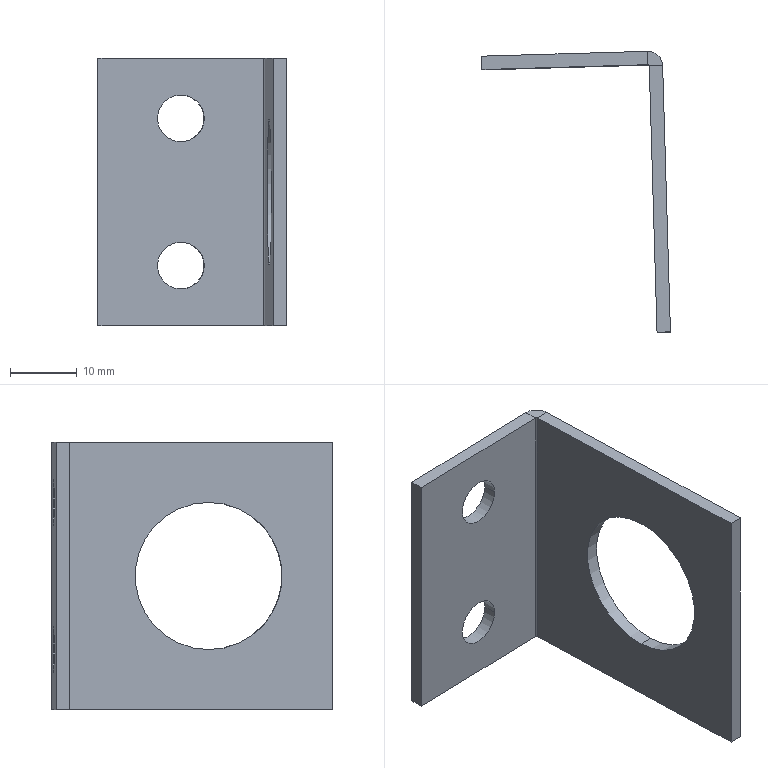Component | SolidWorks | CylinderFixingSheetMetal-1 | 1 solid | 20 faces | box 28.21 x 41.98 x 40 mm | volume 4405 mm3 | plane 12 | cylinder 8 | commonest cylinder face diameters 7 x4 22 x2 4.4 x1 0.4 x1 | material Q235
STEP:
#1=CARTESIAN_POINT('',(-7.163,-7.612,-48.827));
#2=VERTEX_POINT('',#1);
#3=CARTESIAN_POINT('',(-6.887,-7.604,-48.827));
#4=VERTEX_POINT('',#3);
#5=CARTESIAN_POINT('',(-7.025,-7.608,-48.827));
#6=DIRECTION('',(0.02918,-0.9996,-0.));
#7=DIRECTION('',(0.9996,0.02918,0.));
#8=AXIS2_PLACEMENT_3D('',#5,#6,#7);
#9=CIRCLE('',#8,0.1378);
#10=EDGE_CURVE('',#2,#4,#9,.T.);
#11=ORIENTED_EDGE('',*,*,#10,.T.);
#12=CARTESIAN_POINT('',(-6.89,-7.525,-48.827));
#13=VERTEX_POINT('',#12);
#14=CARTESIAN_POINT('',(-6.841,-9.178,-48.827));
#15=DIRECTION('',(-0.02918,0.9996,0.));
#16=VECTOR('',#15,39.37);
#17=LINE('',#14,#16);
#18=EDGE_CURVE('',#4,#13,#17,.T.);
#19=ORIENTED_EDGE('',*,*,#18,.T.);
#20=CARTESIAN_POINT('',(-7.165,-7.533,-48.827));
#21=VERTEX_POINT('',#20);
#22=CARTESIAN_POINT('',(-7.027,-7.529,-48.827));
#23=DIRECTION('',(-0.02918,0.9996,0.));
#24=DIRECTION('',(-0.9996,-0.02918,0.));
#25=AXIS2_PLACEMENT_3D('',#22,#23,#24);
#26=CIRCLE('',#25,0.1378);
#27=EDGE_CURVE('',#13,#21,#26,.T.);
#28=ORIENTED_EDGE('',*,*,#27,.T.);
#29=CARTESIAN_POINT('',(-7.117,-9.186,-48.827));
#30=DIRECTION('',(-0.02918,0.9996,0.));
#31=VECTOR('',#30,39.37);
#32=LINE('',#29,#31);
#33=EDGE_CURVE('',#2,#21,#32,.T.);
#34=ORIENTED_EDGE('',*,*,#33,.F.);
#35=EDGE_LOOP('',(#11,#19,#28,#34));
#36=FACE_OUTER_BOUND('',#35,.T.);
#37=CARTESIAN_POINT('',(-6.979,-9.182,-48.827));
#38=DIRECTION('',(-0.02918,0.9996,0.));
#39=DIRECTION('',(-0.9996,-0.02918,0.));
#40=AXIS2_PLACEMENT_3D('',#37,#38,#39);
#41=CYLINDRICAL_SURFACE('',#40,0.1378);
#42=ADVANCED_FACE('',(#36),#41,.F.);
#43=CARTESIAN_POINT('',(-7.163,-7.612,-47.961));
#44=VERTEX_POINT('',#43);
#45=CARTESIAN_POINT('',(-6.887,-7.604,-47.961));
#46=VERTEX_POINT('',#45);
#47=CARTESIAN_POINT('',(-7.025,-7.608,-47.961));
#48=DIRECTION('',(0.02918,-0.9996,-0.));
#49=DIRECTION('',(0.9996,0.02918,0.));
#50=AXIS2_PLACEMENT_3D('',#47,#48,#49);
#51=CIRCLE('',#50,0.1378);
#52=EDGE_CURVE('',#44,#46,#51,.T.);
#53=ORIENTED_EDGE('',*,*,#52,.T.);
#54=CARTESIAN_POINT('',(-6.89,-7.525,-47.961));
#55=VERTEX_POINT('',#54);
#56=CARTESIAN_POINT('',(-6.841,-9.178,-47.961));
#57=DIRECTION('',(-0.02918,0.9996,0.));
#58=VECTOR('',#57,39.37);
#59=LINE('',#56,#58);
#60=EDGE_CURVE('',#46,#55,#59,.T.);
#61=ORIENTED_EDGE('',*,*,#60,.T.);
#62=CARTESIAN_POINT('',(-7.165,-7.533,-47.961));
#63=VERTEX_POINT('',#62);
#64=CARTESIAN_POINT('',(-7.027,-7.529,-47.961));
#65=DIRECTION('',(-0.02918,0.9996,0.));
#66=DIRECTION('',(-0.9996,-0.02918,0.));
#67=AXIS2_PLACEMENT_3D('',#64,#65,#66);
#68=CIRCLE('',#67,0.1378);
#69=EDGE_CURVE('',#55,#63,#68,.T.);
#70=ORIENTED_EDGE('',*,*,#69,.T.);
#71=CARTESIAN_POINT('',(-7.117,-9.186,-47.961));
#72=DIRECTION('',(-0.02918,0.9996,0.));
#73=VECTOR('',#72,39.37);
#74=LINE('',#71,#73);
#75=EDGE_CURVE('',#44,#63,#74,.T.);
#76=ORIENTED_EDGE('',*,*,#75,.F.);
#77=EDGE_LOOP('',(#53,#61,#70,#76));
#78=FACE_OUTER_BOUND('',#77,.T.);
#79=CARTESIAN_POINT('',(-6.979,-9.182,-47.961));
#80=DIRECTION('',(-0.02918,0.9996,0.));
#81=DIRECTION('',(-0.9996,-0.02918,0.));
#82=AXIS2_PLACEMENT_3D('',#79,#80,#81);
#83=CYLINDRICAL_SURFACE('',#82,0.1378);
#84=ADVANCED_FACE('',(#78),#83,.F.);
#85=CARTESIAN_POINT('',(-6.505,-8.44,-48.827));
#86=VERTEX_POINT('',#85);
#87=CARTESIAN_POINT('',(-6.505,-8.44,-47.961));
#88=VERTEX_POINT('',#87);
#89=CARTESIAN_POINT('',(-6.505,-8.44,-48.394));
#90=DIRECTION('',(-0.9996,-0.02918,0.));
#91=DIRECTION('',(0.,0.,1.));
#92=AXIS2_PLACEMENT_3D('',#89,#90,#91);
#93=CIRCLE('',#92,0.4331);
#94=EDGE_CURVE('',#86,#88,#93,.T.);
#95=ORIENTED_EDGE('',*,*,#94,.T.);
#96=CARTESIAN_POINT('',(-6.426,-8.437,-47.961));
#97=VERTEX_POINT('',#96);
#98=CARTESIAN_POINT('',(-7.488,-8.469,-47.961));
#99=DIRECTION('',(0.9996,0.02918,-0.));
#100=VECTOR('',#99,39.37);
#101=LINE('',#98,#100);
#102=EDGE_CURVE('',#88,#97,#101,.T.);
#103=ORIENTED_EDGE('',*,*,#102,.T.);
#104=CARTESIAN_POINT('',(-6.426,-8.437,-48.827));
#105=VERTEX_POINT('',#104);
#106=CARTESIAN_POINT('',(-6.426,-8.437,-48.394));
#107=DIRECTION('',(0.9996,0.02918,-0.));
#108=DIRECTION('',(-0.,0.,-1.));
#109=AXIS2_PLACEMENT_3D('',#106,#107,#108);
#110=CIRCLE('',#109,0.4331);
#111=EDGE_CURVE('',#97,#105,#110,.T.);
#112=ORIENTED_EDGE('',*,*,#111,.T.);
#113=CARTESIAN_POINT('',(-7.488,-8.469,-48.827));
#114=DIRECTION('',(0.9996,0.02918,-0.));
#115=VECTOR('',#114,39.37);
#116=LINE('',#113,#115);
#117=EDGE_CURVE('',#86,#105,#116,.T.);
#118=ORIENTED_EDGE('',*,*,#117,.F.);
#119=EDGE_LOOP('',(#95,#103,#112,#118));
#120=FACE_OUTER_BOUND('',#119,.T.);
#121=CARTESIAN_POINT('',(-7.488,-8.469,-48.394));
#122=DIRECTION('',(0.9996,0.02918,-0.));
#123=DIRECTION('',(-0.,0.,-1.));
#124=AXIS2_PLACEMENT_3D('',#121,#122,#123);
#125=CYLINDRICAL_SURFACE('',#124,0.4331);
#126=ADVANCED_FACE('',(#120),#125,.F.);
#127=CARTESIAN_POINT('',(-6.529,-7.602,-49.181));
#128=VERTEX_POINT('',#127);
#129=CARTESIAN_POINT('',(-6.483,-9.168,-49.181));
#130=VERTEX_POINT('',#129);
#131=CARTESIAN_POINT('',(-6.529,-7.594,-49.181));
#132=DIRECTION('',(0.02918,-0.9996,-0.));
#133=VECTOR('',#132,39.37);
#134=LINE('',#131,#133);
#135=EDGE_CURVE('',#128,#130,#134,.T.);
#136=ORIENTED_EDGE('',*,*,#135,.F.);
#137=CARTESIAN_POINT('',(-6.45,-7.599,-49.181));
#138=VERTEX_POINT('',#137);
#139=CARTESIAN_POINT('',(-6.529,-7.602,-49.181));
#140=DIRECTION('',(0.9996,0.02918,-0.));
#141=VECTOR('',#140,39.37);
#142=LINE('',#139,#141);
#143=EDGE_CURVE('',#128,#138,#142,.T.);
#144=ORIENTED_EDGE('',*,*,#143,.T.);
#145=CARTESIAN_POINT('',(-6.405,-9.166,-49.181));
#146=VERTEX_POINT('',#145);
#147=CARTESIAN_POINT('',(-6.451,-7.591,-49.181));
#148=DIRECTION('',(0.02918,-0.9996,-0.));
#149=VECTOR('',#148,39.37);
#150=LINE('',#147,#149);
#151=EDGE_CURVE('',#138,#146,#150,.T.);
#152=ORIENTED_EDGE('',*,*,#151,.T.);
#153=CARTESIAN_POINT('',(-6.405,-9.166,-49.181));
#154=DIRECTION('',(-0.9996,-0.02918,0.));
#155=VECTOR('',#154,39.37);
#156=LINE('',#153,#155);
#157=EDGE_CURVE('',#146,#130,#156,.T.);
#158=ORIENTED_EDGE('',*,*,#157,.T.);
#159=EDGE_LOOP('',(#136,#144,#152,#158));
#160=FACE_OUTER_BOUND('',#159,.T.);
#161=CARTESIAN_POINT('',(-6.451,-7.591,-49.181));
#162=DIRECTION('',(-0.,-0.,-1.));
#163=DIRECTION('',(0.02918,-0.9996,-0.));
#164=AXIS2_PLACEMENT_3D('',#161,#162,#163);
#165=PLANE('',#164);
#166=ADVANCED_FACE('',(#160),#165,.T.);
#167=CARTESIAN_POINT('',(-6.426,-8.437,-48.394));
#168=DIRECTION('',(0.9996,0.02918,-0.));
#169=DIRECTION('',(-0.,0.,-1.));
#170=AXIS2_PLACEMENT_3D('',#167,#168,#169);
#171=CIRCLE('',#170,0.4331);
#172=EDGE_CURVE('',#105,#97,#171,.T.);
#173=ORIENTED_EDGE('',*,*,#172,.F.);
#174=ORIENTED_EDGE('',*,*,#111,.F.);
#175=EDGE_LOOP('',(#173,#174));
#176=FACE_BOUND('',#175,.T.);
#177=CARTESIAN_POINT('',(-6.45,-7.599,-47.607));
#178=VERTEX_POINT('',#177);
#179=CARTESIAN_POINT('',(-6.45,-7.599,-49.181));
#180=DIRECTION('',(0.,0.,1.));
#181=VECTOR('',#180,39.37);
#182=LINE('',#179,#181);
#183=EDGE_CURVE('',#138,#178,#182,.T.);
#184=ORIENTED_EDGE('',*,*,#183,.T.);
#185=CARTESIAN_POINT('',(-6.405,-9.166,-47.607));
#186=VERTEX_POINT('',#185);
#187=CARTESIAN_POINT('',(-6.451,-7.591,-47.607));
#188=DIRECTION('',(-0.02918,0.9996,0.));
#189=VECTOR('',#188,39.37);
#190=LINE('',#187,#189);
#191=EDGE_CURVE('',#186,#178,#190,.T.);
#192=ORIENTED_EDGE('',*,*,#191,.F.);
#193=CARTESIAN_POINT('',(-6.405,-9.166,-49.181));
#194=DIRECTION('',(0.,0.,1.));
#195=VECTOR('',#194,39.37);
#196=LINE('',#193,#195);
#197=EDGE_CURVE('',#146,#186,#196,.T.);
#198=ORIENTED_EDGE('',*,*,#197,.F.);
#199=ORIENTED_EDGE('',*,*,#151,.F.);
#200=EDGE_LOOP('',(#184,#192,#198,#199));
#201=FACE_OUTER_BOUND('',#200,.T.);
#202=CARTESIAN_POINT('',(-6.428,-8.378,-48.394));
#203=DIRECTION('',(-0.9996,-0.02918,0.));
#204=DIRECTION('',(0.,0.,1.));
#205=AXIS2_PLACEMENT_3D('',#202,#203,#204);
#206=PLANE('',#205);
#207=ADVANCED_FACE('',(#176,#201),#206,.F.);
#208=ORIENTED_EDGE('',*,*,#94,.F.);
#209=CARTESIAN_POINT('',(-6.505,-8.44,-48.394));
#210=DIRECTION('',(-0.9996,-0.02918,0.));
#211=DIRECTION('',(0.,0.,1.));
#212=AXIS2_PLACEMENT_3D('',#209,#210,#211);
#213=CIRCLE('',#212,0.4331);
#214=EDGE_CURVE('',#88,#86,#213,.T.);
#215=ORIENTED_EDGE('',*,*,#214,.F.);
#216=EDGE_LOOP('',(#208,#215));
#217=FACE_BOUND('',#216,.T.);
#218=CARTESIAN_POINT('',(-6.483,-9.168,-47.607));
#219=VERTEX_POINT('',#218);
#220=CARTESIAN_POINT('',(-6.529,-7.602,-47.607));
#221=VERTEX_POINT('',#220);
#222=CARTESIAN_POINT('',(-6.529,-7.594,-47.607));
#223=DIRECTION('',(-0.02918,0.9996,0.));
#224=VECTOR('',#223,39.37);
#225=LINE('',#222,#224);
#226=EDGE_CURVE('',#219,#221,#225,.T.);
#227=ORIENTED_EDGE('',*,*,#226,.T.);
#228=CARTESIAN_POINT('',(-6.529,-7.602,-49.181));
#229=DIRECTION('',(0.,0.,1.));
#230=VECTOR('',#229,39.37);
#231=LINE('',#228,#230);
#232=EDGE_CURVE('',#128,#221,#231,.T.);
#233=ORIENTED_EDGE('',*,*,#232,.F.);
#234=ORIENTED_EDGE('',*,*,#135,.T.);
#235=CARTESIAN_POINT('',(-6.483,-9.168,-49.181));
#236=DIRECTION('',(0.,0.,1.));
#237=VECTOR('',#236,39.37);
#238=LINE('',#235,#237);
#239=EDGE_CURVE('',#130,#219,#238,.T.);
#240=ORIENTED_EDGE('',*,*,#239,.T.);
#241=EDGE_LOOP('',(#227,#233,#234,#240));
#242=FACE_OUTER_BOUND('',#241,.T.);
#243=CARTESIAN_POINT('',(-6.506,-8.381,-48.394));
#244=DIRECTION('',(-0.9996,-0.02918,0.));
#245=DIRECTION('',(0.,0.,1.));
#246=AXIS2_PLACEMENT_3D('',#243,#244,#245);
#247=PLANE('',#246);
#248=ADVANCED_FACE('',(#217,#242),#247,.T.);
#249=CARTESIAN_POINT('',(-6.529,-7.602,-47.607));
#250=DIRECTION('',(0.9996,0.02918,-0.));
#251=VECTOR('',#250,39.37);
#252=LINE('',#249,#251);
#253=EDGE_CURVE('',#221,#178,#252,.T.);
#254=ORIENTED_EDGE('',*,*,#253,.F.);
#255=ORIENTED_EDGE('',*,*,#226,.F.);
#256=CARTESIAN_POINT('',(-6.405,-9.166,-47.607));
#257=DIRECTION('',(-0.9996,-0.02918,0.));
#258=VECTOR('',#257,39.37);
#259=LINE('',#256,#258);
#260=EDGE_CURVE('',#186,#219,#259,.T.);
#261=ORIENTED_EDGE('',*,*,#260,.F.);
#262=ORIENTED_EDGE('',*,*,#191,.T.);
#263=EDGE_LOOP('',(#254,#255,#261,#262));
#264=FACE_OUTER_BOUND('',#263,.T.);
#265=CARTESIAN_POINT('',(-6.451,-7.591,-47.607));
#266=DIRECTION('',(0.,0.,1.));
#267=DIRECTION('',(0.9996,0.02918,-0.));
#268=AXIS2_PLACEMENT_3D('',#265,#266,#267);
#269=PLANE('',#268);
#270=ADVANCED_FACE('',(#264),#269,.T.);
#271=ORIENTED_EDGE('',*,*,#239,.F.);
#272=ORIENTED_EDGE('',*,*,#157,.F.);
#273=ORIENTED_EDGE('',*,*,#197,.T.);
#274=ORIENTED_EDGE('',*,*,#260,.T.);
#275=EDGE_LOOP('',(#271,#272,#273,#274));
#276=FACE_OUTER_BOUND('',#275,.T.);
#277=CARTESIAN_POINT('',(-6.405,-9.166,-49.181));
#278=DIRECTION('',(0.02918,-0.9996,-0.));
#279=DIRECTION('',(0.9996,0.02918,-0.));
#280=AXIS2_PLACEMENT_3D('',#277,#278,#279);
#281=PLANE('',#280);
#282=ADVANCED_FACE('',(#276),#281,.T.);
#283=CARTESIAN_POINT('',(-6.537,-7.594,-47.607));
#284=VERTEX_POINT('',#283);
#285=CARTESIAN_POINT('',(-6.539,-7.515,-47.607));
#286=VERTEX_POINT('',#285);
#287=CARTESIAN_POINT('',(-6.537,-7.594,-47.607));
#288=DIRECTION('',(-0.02918,0.9996,0.));
#289=VECTOR('',#288,39.37);
#290=LINE('',#287,#289);
#291=EDGE_CURVE('',#284,#286,#290,.T.);
#292=ORIENTED_EDGE('',*,*,#291,.F.);
#293=CARTESIAN_POINT('',(-6.537,-7.602,-47.607));
#294=DIRECTION('',(0.,0.,1.));
#295=DIRECTION('',(-0.9996,-0.02918,0.));
#296=AXIS2_PLACEMENT_3D('',#293,#294,#295);
#297=CIRCLE('',#296,0.007874);
#298=EDGE_CURVE('',#221,#284,#297,.T.);
#299=ORIENTED_EDGE('',*,*,#298,.F.);
#300=ORIENTED_EDGE('',*,*,#253,.T.);
#301=CARTESIAN_POINT('',(-6.537,-7.602,-47.607));
#302=DIRECTION('',(0.,0.,1.));
#303=DIRECTION('',(-0.9996,-0.02918,0.));
#304=AXIS2_PLACEMENT_3D('',#301,#302,#303);
#305=CIRCLE('',#304,0.08661);
#306=EDGE_CURVE('',#178,#286,#305,.T.);
#307=ORIENTED_EDGE('',*,*,#306,.T.);
#308=EDGE_LOOP('',(#292,#299,#300,#307));
#309=FACE_OUTER_BOUND('',#308,.T.);
#310=CARTESIAN_POINT('',(-6.537,-7.602,-47.607));
#311=DIRECTION('',(0.,0.,1.));
#312=DIRECTION('',(0.9996,0.02918,-0.));
#313=AXIS2_PLACEMENT_3D('',#310,#311,#312);
#314=PLANE('',#313);
#315=ADVANCED_FACE('',(#309),#314,.T.);
#316=CARTESIAN_POINT('',(-6.537,-7.594,-49.181));
#317=VERTEX_POINT('',#316);
#318=CARTESIAN_POINT('',(-6.537,-7.602,-49.181));
#319=DIRECTION('',(-0.,-0.,-1.));
#320=DIRECTION('',(-0.9996,-0.02918,0.));
#321=AXIS2_PLACEMENT_3D('',#318,#319,#320);
#322=CIRCLE('',#321,0.007874);
#323=EDGE_CURVE('',#317,#128,#322,.T.);
#324=ORIENTED_EDGE('',*,*,#323,.F.);
#325=CARTESIAN_POINT('',(-6.539,-7.515,-49.181));
#326=VERTEX_POINT('',#325);
#327=CARTESIAN_POINT('',(-6.537,-7.594,-49.181));
#328=DIRECTION('',(-0.02918,0.9996,0.));
#329=VECTOR('',#328,39.37);
#330=LINE('',#327,#329);
#331=EDGE_CURVE('',#317,#326,#330,.T.);
#332=ORIENTED_EDGE('',*,*,#331,.T.);
#333=CARTESIAN_POINT('',(-6.537,-7.602,-49.181));
#334=DIRECTION('',(-0.,-0.,-1.));
#335=DIRECTION('',(-0.9996,-0.02918,0.));
#336=AXIS2_PLACEMENT_3D('',#333,#334,#335);
#337=CIRCLE('',#336,0.08661);
#338=EDGE_CURVE('',#326,#138,#337,.T.);
#339=ORIENTED_EDGE('',*,*,#338,.T.);
#340=ORIENTED_EDGE('',*,*,#143,.F.);
#341=EDGE_LOOP('',(#324,#332,#339,#340));
#342=FACE_OUTER_BOUND('',#341,.T.);
#343=CARTESIAN_POINT('',(-6.537,-7.602,-49.181));
#344=DIRECTION('',(0.,0.,1.));
#345=DIRECTION('',(0.9996,0.02918,-0.));
#346=AXIS2_PLACEMENT_3D('',#343,#344,#345);
#347=PLANE('',#346);
#348=ADVANCED_FACE('',(#342),#347,.F.);
#349=ORIENTED_EDGE('',*,*,#183,.F.);
#350=ORIENTED_EDGE('',*,*,#338,.F.);
#351=CARTESIAN_POINT('',(-6.539,-7.515,-48.394));
#352=DIRECTION('',(0.,0.,1.));
#353=VECTOR('',#352,39.37);
#354=LINE('',#351,#353);
#355=EDGE_CURVE('',#326,#286,#354,.T.);
#356=ORIENTED_EDGE('',*,*,#355,.T.);
#357=ORIENTED_EDGE('',*,*,#306,.F.);
#358=EDGE_LOOP('',(#349,#350,#356,#357));
#359=FACE_OUTER_BOUND('',#358,.T.);
#360=CARTESIAN_POINT('',(-6.537,-7.602,-49.181));
#361=DIRECTION('',(-0.,-0.,-1.));
#362=DIRECTION('',(-0.02918,0.9996,0.));
#363=AXIS2_PLACEMENT_3D('',#360,#361,#362);
#364=CYLINDRICAL_SURFACE('',#363,0.08661);
#365=ADVANCED_FACE('',(#359),#364,.T.);
#366=ORIENTED_EDGE('',*,*,#232,.T.);
#367=ORIENTED_EDGE('',*,*,#298,.T.);
#368=CARTESIAN_POINT('',(-6.537,-7.594,-47.607));
#369=DIRECTION('',(-0.,-0.,-1.));
#370=VECTOR('',#369,39.37);
#371=LINE('',#368,#370);
#372=EDGE_CURVE('',#284,#317,#371,.T.);
#373=ORIENTED_EDGE('',*,*,#372,.T.);
#374=ORIENTED_EDGE('',*,*,#323,.T.);
#375=EDGE_LOOP('',(#366,#367,#373,#374));
#376=FACE_OUTER_BOUND('',#375,.T.);
#377=CARTESIAN_POINT('',(-6.537,-7.602,-49.181));
#378=DIRECTION('',(-0.,-0.,-1.));
#379=DIRECTION('',(-0.02918,0.9996,0.));
#380=AXIS2_PLACEMENT_3D('',#377,#378,#379);
#381=CYLINDRICAL_SURFACE('',#380,0.007874);
#382=ADVANCED_FACE('',(#376),#381,.F.);
#383=ORIENTED_EDGE('',*,*,#291,.T.);
#384=CARTESIAN_POINT('',(-7.515,-7.544,-47.607));
#385=VERTEX_POINT('',#384);
#386=CARTESIAN_POINT('',(-6.532,-7.515,-47.607));
#387=DIRECTION('',(0.9996,0.02918,-0.));
#388=VECTOR('',#387,39.37);
#389=LINE('',#386,#388);
#390=EDGE_CURVE('',#385,#286,#389,.T.);
#391=ORIENTED_EDGE('',*,*,#390,.F.);
#392=CARTESIAN_POINT('',(-7.513,-7.622,-47.607));
#393=VERTEX_POINT('',#392);
#394=CARTESIAN_POINT('',(-7.515,-7.544,-47.607));
#395=DIRECTION('',(0.02918,-0.9996,-0.));
#396=VECTOR('',#395,39.37);
#397=LINE('',#394,#396);
#398=EDGE_CURVE('',#385,#393,#397,.T.);
#399=ORIENTED_EDGE('',*,*,#398,.T.);
#400=CARTESIAN_POINT('',(-6.529,-7.594,-47.607));
#401=DIRECTION('',(0.9996,0.02918,-0.));
#402=VECTOR('',#401,39.37);
#403=LINE('',#400,#402);
#404=EDGE_CURVE('',#393,#284,#403,.T.);
#405=ORIENTED_EDGE('',*,*,#404,.T.);
#406=EDGE_LOOP('',(#383,#391,#399,#405));
#407=FACE_OUTER_BOUND('',#406,.T.);
#408=CARTESIAN_POINT('',(-6.532,-7.515,-47.607));
#409=DIRECTION('',(-0.,-0.,-1.));
#410=DIRECTION('',(-0.9996,-0.02918,0.));
#411=AXIS2_PLACEMENT_3D('',#408,#409,#410);
#412=PLANE('',#411);
#413=ADVANCED_FACE('',(#407),#412,.F.);
#414=ORIENTED_EDGE('',*,*,#331,.F.);
#415=CARTESIAN_POINT('',(-7.513,-7.622,-49.181));
#416=VERTEX_POINT('',#415);
#417=CARTESIAN_POINT('',(-7.513,-7.622,-49.181));
#418=DIRECTION('',(-0.9996,-0.02918,0.));
#419=VECTOR('',#418,39.37);
#420=LINE('',#417,#419);
#421=EDGE_CURVE('',#317,#416,#420,.T.);
#422=ORIENTED_EDGE('',*,*,#421,.T.);
#423=CARTESIAN_POINT('',(-7.515,-7.544,-49.181));
#424=VERTEX_POINT('',#423);
#425=CARTESIAN_POINT('',(-7.515,-7.544,-49.181));
#426=DIRECTION('',(0.02918,-0.9996,-0.));
#427=VECTOR('',#426,39.37);
#428=LINE('',#425,#427);
#429=EDGE_CURVE('',#424,#416,#428,.T.);
#430=ORIENTED_EDGE('',*,*,#429,.F.);
#431=CARTESIAN_POINT('',(-7.515,-7.544,-49.181));
#432=DIRECTION('',(-0.9996,-0.02918,0.));
#433=VECTOR('',#432,39.37);
#434=LINE('',#431,#433);
#435=EDGE_CURVE('',#326,#424,#434,.T.);
#436=ORIENTED_EDGE('',*,*,#435,.F.);
#437=EDGE_LOOP('',(#414,#422,#430,#436));
#438=FACE_OUTER_BOUND('',#437,.T.);
#439=CARTESIAN_POINT('',(-7.515,-7.544,-49.181));
#440=DIRECTION('',(0.,0.,1.));
#441=DIRECTION('',(0.9996,0.02918,-0.));
#442=AXIS2_PLACEMENT_3D('',#439,#440,#441);
#443=PLANE('',#442);
#444=ADVANCED_FACE('',(#438),#443,.F.);
#445=CARTESIAN_POINT('',(-7.027,-7.529,-48.827));
#446=DIRECTION('',(-0.02918,0.9996,0.));
#447=DIRECTION('',(-0.9996,-0.02918,0.));
#448=AXIS2_PLACEMENT_3D('',#445,#446,#447);
#449=CIRCLE('',#448,0.1378);
#450=EDGE_CURVE('',#21,#13,#449,.T.);
#451=ORIENTED_EDGE('',*,*,#450,.F.);
#452=ORIENTED_EDGE('',*,*,#27,.F.);
#453=EDGE_LOOP('',(#451,#452));
#454=FACE_BOUND('',#453,.T.);
#455=CARTESIAN_POINT('',(-7.027,-7.529,-47.961));
#456=DIRECTION('',(-0.02918,0.9996,0.));
#457=DIRECTION('',(-0.9996,-0.02918,0.));
#458=AXIS2_PLACEMENT_3D('',#455,#456,#457);
#459=CIRCLE('',#458,0.1378);
#460=EDGE_CURVE('',#63,#55,#459,.T.);
#461=ORIENTED_EDGE('',*,*,#460,.F.);
#462=ORIENTED_EDGE('',*,*,#69,.F.);
#463=EDGE_LOOP('',(#461,#462));
#464=FACE_BOUND('',#463,.T.);
#465=ORIENTED_EDGE('',*,*,#355,.F.);
#466=ORIENTED_EDGE('',*,*,#435,.T.);
#467=CARTESIAN_POINT('',(-7.515,-7.544,-47.607));
#468=DIRECTION('',(0.,0.,1.));
#469=VECTOR('',#468,39.37);
#470=LINE('',#467,#469);
#471=EDGE_CURVE('',#424,#385,#470,.T.);
#472=ORIENTED_EDGE('',*,*,#471,.T.);
#473=ORIENTED_EDGE('',*,*,#390,.T.);
#474=EDGE_LOOP('',(#465,#466,#472,#473));
#475=FACE_OUTER_BOUND('',#474,.T.);
#476=CARTESIAN_POINT('',(-6.532,-7.515,-48.394));
#477=DIRECTION('',(0.02918,-0.9996,-0.));
#478=DIRECTION('',(0.9996,0.02918,-0.));
#479=AXIS2_PLACEMENT_3D('',#476,#477,#478);
#480=PLANE('',#479);
#481=ADVANCED_FACE('',(#454,#464,#475),#480,.F.);
#482=ORIENTED_EDGE('',*,*,#10,.F.);
#483=CARTESIAN_POINT('',(-7.025,-7.608,-48.827));
#484=DIRECTION('',(0.02918,-0.9996,-0.));
#485=DIRECTION('',(0.9996,0.02918,0.));
#486=AXIS2_PLACEMENT_3D('',#483,#484,#485);
#487=CIRCLE('',#486,0.1378);
#488=EDGE_CURVE('',#4,#2,#487,.T.);
#489=ORIENTED_EDGE('',*,*,#488,.F.);
#490=EDGE_LOOP('',(#482,#489));
#491=FACE_BOUND('',#490,.T.);
#492=ORIENTED_EDGE('',*,*,#52,.F.);
#493=CARTESIAN_POINT('',(-7.025,-7.608,-47.961));
#494=DIRECTION('',(0.02918,-0.9996,-0.));
#495=DIRECTION('',(0.9996,0.02918,0.));
#496=AXIS2_PLACEMENT_3D('',#493,#494,#495);
#497=CIRCLE('',#496,0.1378);
#498=EDGE_CURVE('',#46,#44,#497,.T.);
#499=ORIENTED_EDGE('',*,*,#498,.F.);
#500=EDGE_LOOP('',(#492,#499));
#501=FACE_BOUND('',#500,.T.);
#502=ORIENTED_EDGE('',*,*,#421,.F.);
#503=ORIENTED_EDGE('',*,*,#372,.F.);
#504=ORIENTED_EDGE('',*,*,#404,.F.);
#505=CARTESIAN_POINT('',(-7.513,-7.622,-47.607));
#506=DIRECTION('',(0.,0.,1.));
#507=VECTOR('',#506,39.37);
#508=LINE('',#505,#507);
#509=EDGE_CURVE('',#416,#393,#508,.T.);
#510=ORIENTED_EDGE('',*,*,#509,.F.);
#511=EDGE_LOOP('',(#502,#503,#504,#510));
#512=FACE_OUTER_BOUND('',#511,.T.);
#513=CARTESIAN_POINT('',(-6.529,-7.594,-48.394));
#514=DIRECTION('',(0.02918,-0.9996,-0.));
#515=DIRECTION('',(0.9996,0.02918,-0.));
#516=AXIS2_PLACEMENT_3D('',#513,#514,#515);
#517=PLANE('',#516);
#518=ADVANCED_FACE('',(#491,#501,#512),#517,.T.);
#519=ORIENTED_EDGE('',*,*,#509,.T.);
#520=ORIENTED_EDGE('',*,*,#398,.F.);
#521=ORIENTED_EDGE('',*,*,#471,.F.);
#522=ORIENTED_EDGE('',*,*,#429,.T.);
#523=EDGE_LOOP('',(#519,#520,#521,#522));
#524=FACE_OUTER_BOUND('',#523,.T.);
#525=CARTESIAN_POINT('',(-7.515,-7.544,-47.607));
#526=DIRECTION('',(0.9996,0.02918,-0.));
#527=DIRECTION('',(-0.02918,0.9996,0.));
#528=AXIS2_PLACEMENT_3D('',#525,#526,#527);
#529=PLANE('',#528);
#530=ADVANCED_FACE('',(#524),#529,.F.);
#531=ORIENTED_EDGE('',*,*,#102,.F.);
#532=ORIENTED_EDGE('',*,*,#214,.T.);
#533=ORIENTED_EDGE('',*,*,#117,.T.);
#534=ORIENTED_EDGE('',*,*,#172,.T.);
#535=EDGE_LOOP('',(#531,#532,#533,#534));
#536=FACE_OUTER_BOUND('',#535,.T.);
#537=CARTESIAN_POINT('',(-7.488,-8.469,-48.394));
#538=DIRECTION('',(0.9996,0.02918,-0.));
#539=DIRECTION('',(-0.,0.,-1.));
#540=AXIS2_PLACEMENT_3D('',#537,#538,#539);
#541=CYLINDRICAL_SURFACE('',#540,0.4331);
#542=ADVANCED_FACE('',(#536),#541,.F.);
#543=ORIENTED_EDGE('',*,*,#60,.F.);
#544=ORIENTED_EDGE('',*,*,#498,.T.);
#545=ORIENTED_EDGE('',*,*,#75,.T.);
#546=ORIENTED_EDGE('',*,*,#460,.T.);
#547=EDGE_LOOP('',(#543,#544,#545,#546));
#548=FACE_OUTER_BOUND('',#547,.T.);
#549=CARTESIAN_POINT('',(-6.979,-9.182,-47.961));
#550=DIRECTION('',(-0.02918,0.9996,0.));
#551=DIRECTION('',(-0.9996,-0.02918,0.));
#552=AXIS2_PLACEMENT_3D('',#549,#550,#551);
#553=CYLINDRICAL_SURFACE('',#552,0.1378);
#554=ADVANCED_FACE('',(#548),#553,.F.);
#555=ORIENTED_EDGE('',*,*,#18,.F.);
#556=ORIENTED_EDGE('',*,*,#488,.T.);
#557=ORIENTED_EDGE('',*,*,#33,.T.);
#558=ORIENTED_EDGE('',*,*,#450,.T.);
#559=EDGE_LOOP('',(#555,#556,#557,#558));
#560=FACE_OUTER_BOUND('',#559,.T.);
#561=CARTESIAN_POINT('',(-6.979,-9.182,-48.827));
#562=DIRECTION('',(-0.02918,0.9996,0.));
#563=DIRECTION('',(-0.9996,-0.02918,0.));
#564=AXIS2_PLACEMENT_3D('',#561,#562,#563);
#565=CYLINDRICAL_SURFACE('',#564,0.1378);
#566=ADVANCED_FACE('',(#560),#565,.F.);
#567=CLOSED_SHELL('',(#42,#84,#126,#166,#207,#248,#270,#282,#315,#348,#365,#382,#413,#444,#481,#518,#530,#542,#554,#566));
#568=MANIFOLD_SOLID_BREP('',#567);
#569=CARTESIAN_POINT('',(0.,0.,0.));
#570=DIRECTION('',(0.,0.,1.));
#571=DIRECTION('',(1.,0.,0.));
#572=AXIS2_PLACEMENT_3D('',#569,#570,#571);
#573=(LENGTH_UNIT()NAMED_UNIT(*)SI_UNIT($,.METRE.));
#574=LENGTH_MEASURE_WITH_UNIT(LENGTH_MEASURE(0.0254),#573);
#575=DIMENSIONAL_EXPONENTS(1.,0.,0.,0.,0.,0.,0.);
#576=(CONVERSION_BASED_UNIT('',#574)LENGTH_UNIT()NAMED_UNIT(#575));
#577=UNCERTAINTY_MEASURE_WITH_UNIT(LENGTH_MEASURE(0.00001),#576,'','');
#578=(NAMED_UNIT(*)PLANE_ANGLE_UNIT()SI_UNIT($,.RADIAN.));
#579=(NAMED_UNIT(*)SI_UNIT($,.STERADIAN.)SOLID_ANGLE_UNIT());
#580=(GEOMETRIC_REPRESENTATION_CONTEXT(3)GLOBAL_UNCERTAINTY_ASSIGNED_CONTEXT((#577))GLOBAL_UNIT_ASSIGNED_CONTEXT((#576,#578,#579))REPRESENTATION_CONTEXT('',''));
#581=ADVANCED_BREP_SHAPE_REPRESENTATION('',(#568,#572),#580);
#582=COLOUR_RGB('',0.7922,0.8196,0.9333);
#583=FILL_AREA_STYLE_COLOUR('',#582);
#584=FILL_AREA_STYLE('',(#583));
#585=SURFACE_STYLE_FILL_AREA(#584);
#586=SURFACE_SIDE_STYLE('',(#585));
#587=SURFACE_STYLE_USAGE(.BOTH.,#586);
#588=PRESENTATION_STYLE_ASSIGNMENT((#587));
#589=STYLED_ITEM('',(#588),#568);
#590=(LENGTH_UNIT()NAMED_UNIT(*)SI_UNIT($,.METRE.));
#591=LENGTH_MEASURE_WITH_UNIT(LENGTH_MEASURE(0.0254),#590);
#592=DIMENSIONAL_EXPONENTS(1.,0.,0.,0.,0.,0.,0.);
#593=(CONVERSION_BASED_UNIT('',#591)LENGTH_UNIT()NAMED_UNIT(#592));
#594=UNCERTAINTY_MEASURE_WITH_UNIT(LENGTH_MEASURE(0.00001),#593,'','');
#595=(NAMED_UNIT(*)PLANE_ANGLE_UNIT()SI_UNIT($,.RADIAN.));
#596=(NAMED_UNIT(*)SI_UNIT($,.STERADIAN.)SOLID_ANGLE_UNIT());
#597=(GEOMETRIC_REPRESENTATION_CONTEXT(3)GLOBAL_UNCERTAINTY_ASSIGNED_CONTEXT((#594))GLOBAL_UNIT_ASSIGNED_CONTEXT((#593,#595,#596))REPRESENTATION_CONTEXT('',''));
#598=MECHANICAL_DESIGN_GEOMETRIC_PRESENTATION_REPRESENTATION('',(#589),#597);
#599=PRESENTATION_LAYER_ASSIGNMENT('','',(#589));